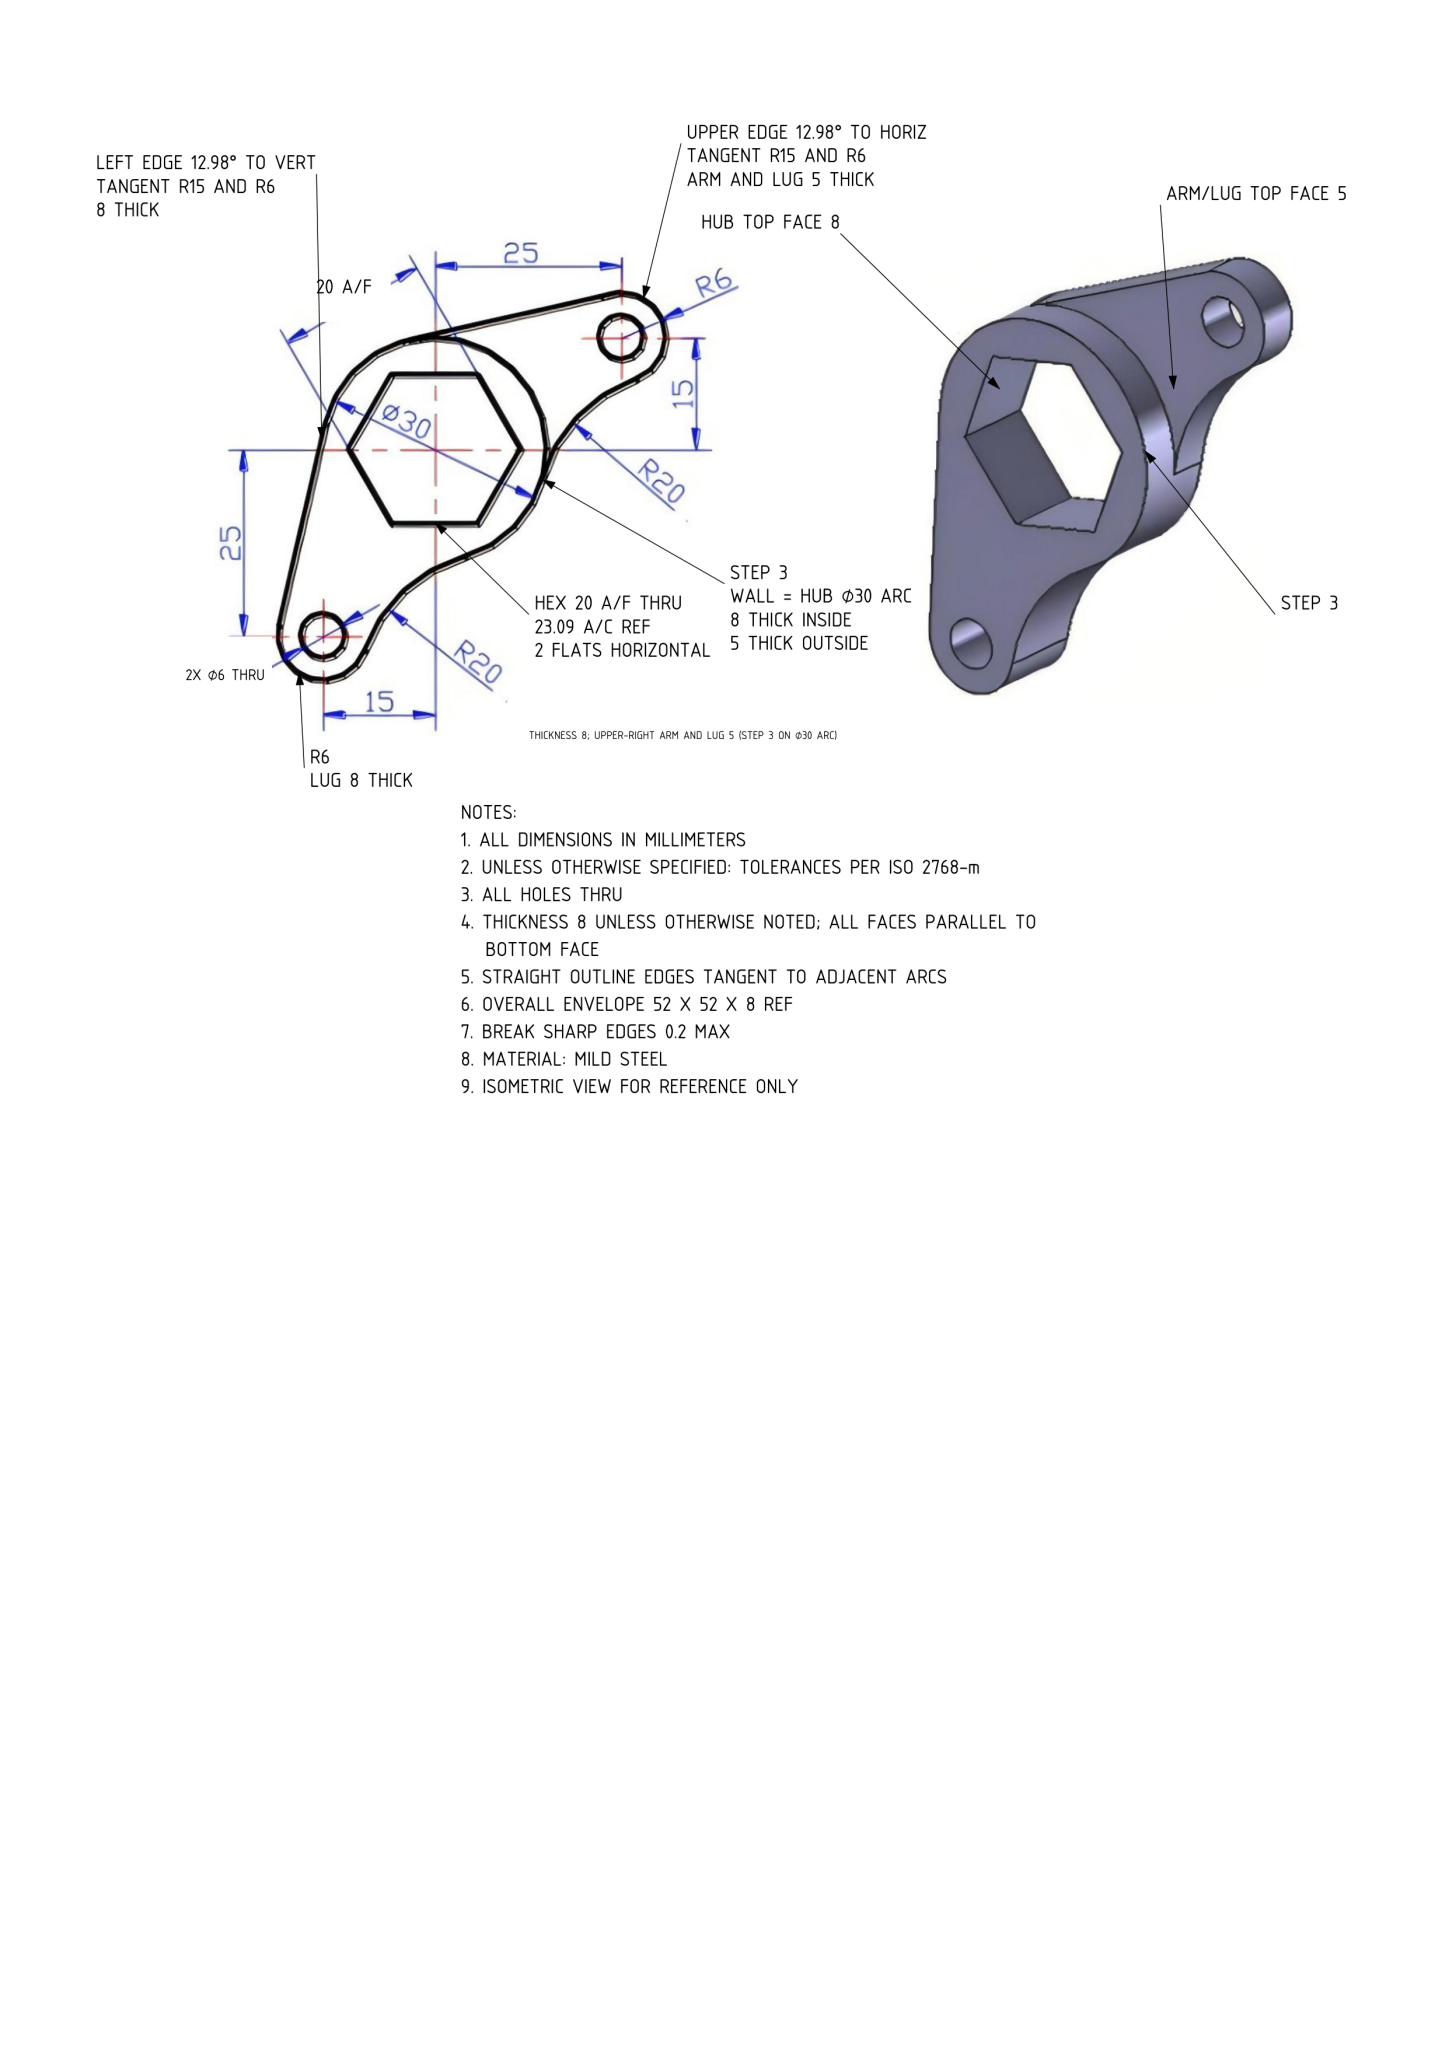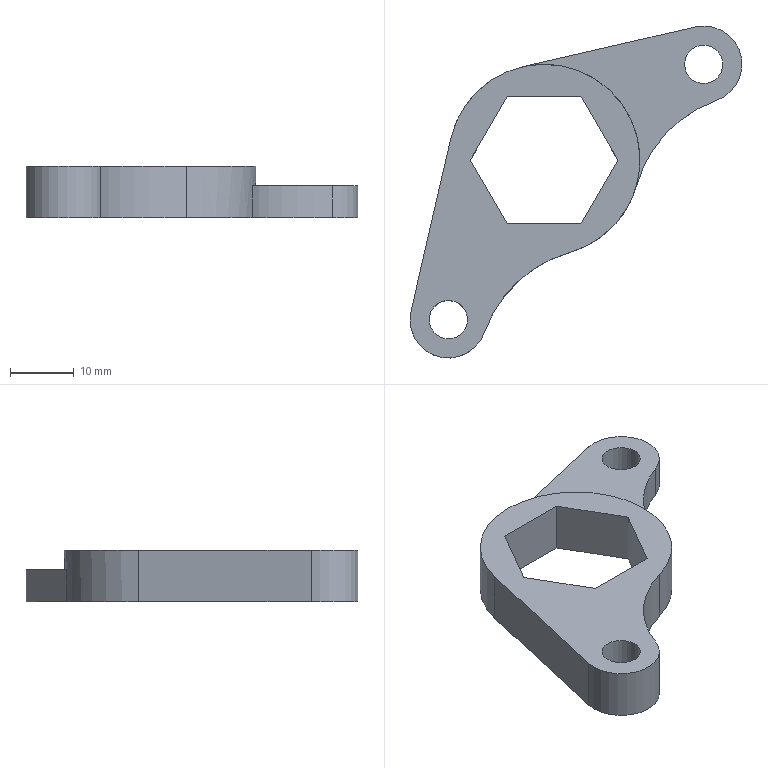Part | NX | mm | 1 solid | 18 faces | box 52 x 52 x 8 mm | volume 6324 mm3 | plane 11 | cylinder 7 | commonest cylinder face diameters 40 x2 12 x2 6 x2 30 x1
STEP:
#1=CARTESIAN_POINT('',(0.,0.,0.));
#2=DIRECTION('',(0.,0.,1.));
#3=DIRECTION('',(1.,0.,0.));
#4=AXIS2_PLACEMENT_3D('',#1,#2,#3);
#5=(LENGTH_UNIT()NAMED_UNIT(*)SI_UNIT(.MILLI.,.METRE.));
#6=UNCERTAINTY_MEASURE_WITH_UNIT(LENGTH_MEASURE(0.00002),#5,'','');
#7=(NAMED_UNIT(*)PLANE_ANGLE_UNIT()SI_UNIT($,.RADIAN.));
#8=PLANE_ANGLE_MEASURE_WITH_UNIT(PLANE_ANGLE_MEASURE(0.01745),#7);
#9=DIMENSIONAL_EXPONENTS(0.,0.,0.,0.,0.,0.,0.);
#10=(CONVERSION_BASED_UNIT('',#8)NAMED_UNIT(#9)PLANE_ANGLE_UNIT());
#11=(NAMED_UNIT(*)SI_UNIT($,.STERADIAN.)SOLID_ANGLE_UNIT());
#12=(GEOMETRIC_REPRESENTATION_CONTEXT(3)GLOBAL_UNCERTAINTY_ASSIGNED_CONTEXT((#6))GLOBAL_UNIT_ASSIGNED_CONTEXT((#5,#10,#11))REPRESENTATION_CONTEXT('',''));
#13=SHAPE_REPRESENTATION('',(#4),#12);
#14=CARTESIAN_POINT('',(-11.547,0.,0.));
#15=VERTEX_POINT('',#14);
#16=CARTESIAN_POINT('',(-5.774,-10.,0.));
#17=VERTEX_POINT('',#16);
#18=CARTESIAN_POINT('',(-11.547,0.,0.));
#19=DIRECTION('',(0.5,-0.866,0.));
#20=VECTOR('',#19,1.);
#21=LINE('',#18,#20);
#22=EDGE_CURVE('',#15,#17,#21,.T.);
#23=ORIENTED_EDGE('',*,*,#22,.F.);
#24=CARTESIAN_POINT('',(-11.547,0.,8.));
#25=VERTEX_POINT('',#24);
#26=CARTESIAN_POINT('',(-11.547,0.,8.));
#27=DIRECTION('',(0.,0.,-1.));
#28=VECTOR('',#27,1.);
#29=LINE('',#26,#28);
#30=EDGE_CURVE('',#25,#15,#29,.T.);
#31=ORIENTED_EDGE('',*,*,#30,.F.);
#32=CARTESIAN_POINT('',(-5.774,-10.,8.));
#33=VERTEX_POINT('',#32);
#34=CARTESIAN_POINT('',(-11.547,0.,8.));
#35=DIRECTION('',(0.5,-0.866,0.));
#36=VECTOR('',#35,1.);
#37=LINE('',#34,#36);
#38=EDGE_CURVE('',#25,#33,#37,.T.);
#39=ORIENTED_EDGE('',*,*,#38,.T.);
#40=CARTESIAN_POINT('',(-5.774,-10.,8.));
#41=DIRECTION('',(0.,0.,-1.));
#42=VECTOR('',#41,1.);
#43=LINE('',#40,#42);
#44=EDGE_CURVE('',#33,#17,#43,.T.);
#45=ORIENTED_EDGE('',*,*,#44,.T.);
#46=EDGE_LOOP('',(#23,#31,#39,#45));
#47=FACE_OUTER_BOUND('',#46,.T.);
#48=CARTESIAN_POINT('',(-11.547,0.,8.));
#49=DIRECTION('',(0.866,0.5,0.));
#50=DIRECTION('',(-0.5,0.866,0.));
#51=AXIS2_PLACEMENT_3D('',#48,#49,#50);
#52=PLANE('',#51);
#53=ADVANCED_FACE('',(#47),#52,.T.);
#54=CARTESIAN_POINT('',(5.774,-10.,0.));
#55=VERTEX_POINT('',#54);
#56=CARTESIAN_POINT('',(-5.774,-10.,0.));
#57=DIRECTION('',(1.,-0.,0.));
#58=VECTOR('',#57,1.);
#59=LINE('',#56,#58);
#60=EDGE_CURVE('',#17,#55,#59,.T.);
#61=ORIENTED_EDGE('',*,*,#60,.F.);
#62=ORIENTED_EDGE('',*,*,#44,.F.);
#63=CARTESIAN_POINT('',(5.774,-10.,8.));
#64=VERTEX_POINT('',#63);
#65=CARTESIAN_POINT('',(-5.774,-10.,8.));
#66=DIRECTION('',(1.,-0.,0.));
#67=VECTOR('',#66,1.);
#68=LINE('',#65,#67);
#69=EDGE_CURVE('',#33,#64,#68,.T.);
#70=ORIENTED_EDGE('',*,*,#69,.T.);
#71=CARTESIAN_POINT('',(5.774,-10.,8.));
#72=DIRECTION('',(0.,0.,-1.));
#73=VECTOR('',#72,1.);
#74=LINE('',#71,#73);
#75=EDGE_CURVE('',#64,#55,#74,.T.);
#76=ORIENTED_EDGE('',*,*,#75,.T.);
#77=EDGE_LOOP('',(#61,#62,#70,#76));
#78=FACE_OUTER_BOUND('',#77,.T.);
#79=CARTESIAN_POINT('',(-5.774,-10.,8.));
#80=DIRECTION('',(0.,1.,0.));
#81=DIRECTION('',(-1.,0.,0.));
#82=AXIS2_PLACEMENT_3D('',#79,#80,#81);
#83=PLANE('',#82);
#84=ADVANCED_FACE('',(#78),#83,.T.);
#85=CARTESIAN_POINT('',(11.547,-0.,0.));
#86=VERTEX_POINT('',#85);
#87=CARTESIAN_POINT('',(5.774,-10.,0.));
#88=DIRECTION('',(0.5,0.866,0.));
#89=VECTOR('',#88,1.);
#90=LINE('',#87,#89);
#91=EDGE_CURVE('',#55,#86,#90,.T.);
#92=ORIENTED_EDGE('',*,*,#91,.F.);
#93=ORIENTED_EDGE('',*,*,#75,.F.);
#94=CARTESIAN_POINT('',(11.547,-0.,8.));
#95=VERTEX_POINT('',#94);
#96=CARTESIAN_POINT('',(5.774,-10.,8.));
#97=DIRECTION('',(0.5,0.866,0.));
#98=VECTOR('',#97,1.);
#99=LINE('',#96,#98);
#100=EDGE_CURVE('',#64,#95,#99,.T.);
#101=ORIENTED_EDGE('',*,*,#100,.T.);
#102=CARTESIAN_POINT('',(11.547,-0.,8.));
#103=DIRECTION('',(0.,0.,-1.));
#104=VECTOR('',#103,1.);
#105=LINE('',#102,#104);
#106=EDGE_CURVE('',#95,#86,#105,.T.);
#107=ORIENTED_EDGE('',*,*,#106,.T.);
#108=EDGE_LOOP('',(#92,#93,#101,#107));
#109=FACE_OUTER_BOUND('',#108,.T.);
#110=CARTESIAN_POINT('',(5.774,-10.,8.));
#111=DIRECTION('',(-0.866,0.5,0.));
#112=DIRECTION('',(-0.5,-0.866,0.));
#113=AXIS2_PLACEMENT_3D('',#110,#111,#112);
#114=PLANE('',#113);
#115=ADVANCED_FACE('',(#109),#114,.T.);
#116=CARTESIAN_POINT('',(5.774,10.,0.));
#117=VERTEX_POINT('',#116);
#118=CARTESIAN_POINT('',(11.547,-0.,0.));
#119=DIRECTION('',(-0.5,0.866,0.));
#120=VECTOR('',#119,1.);
#121=LINE('',#118,#120);
#122=EDGE_CURVE('',#86,#117,#121,.T.);
#123=ORIENTED_EDGE('',*,*,#122,.F.);
#124=ORIENTED_EDGE('',*,*,#106,.F.);
#125=CARTESIAN_POINT('',(5.774,10.,8.));
#126=VERTEX_POINT('',#125);
#127=CARTESIAN_POINT('',(11.547,-0.,8.));
#128=DIRECTION('',(-0.5,0.866,0.));
#129=VECTOR('',#128,1.);
#130=LINE('',#127,#129);
#131=EDGE_CURVE('',#95,#126,#130,.T.);
#132=ORIENTED_EDGE('',*,*,#131,.T.);
#133=CARTESIAN_POINT('',(5.774,10.,8.));
#134=DIRECTION('',(0.,0.,-1.));
#135=VECTOR('',#134,1.);
#136=LINE('',#133,#135);
#137=EDGE_CURVE('',#126,#117,#136,.T.);
#138=ORIENTED_EDGE('',*,*,#137,.T.);
#139=EDGE_LOOP('',(#123,#124,#132,#138));
#140=FACE_OUTER_BOUND('',#139,.T.);
#141=CARTESIAN_POINT('',(11.547,-0.,8.));
#142=DIRECTION('',(-0.866,-0.5,0.));
#143=DIRECTION('',(0.5,-0.866,0.));
#144=AXIS2_PLACEMENT_3D('',#141,#142,#143);
#145=PLANE('',#144);
#146=ADVANCED_FACE('',(#140),#145,.T.);
#147=CARTESIAN_POINT('',(-5.774,10.,0.));
#148=VERTEX_POINT('',#147);
#149=CARTESIAN_POINT('',(5.774,10.,0.));
#150=DIRECTION('',(-1.,0.,0.));
#151=VECTOR('',#150,1.);
#152=LINE('',#149,#151);
#153=EDGE_CURVE('',#117,#148,#152,.T.);
#154=ORIENTED_EDGE('',*,*,#153,.F.);
#155=ORIENTED_EDGE('',*,*,#137,.F.);
#156=CARTESIAN_POINT('',(-5.774,10.,8.));
#157=VERTEX_POINT('',#156);
#158=CARTESIAN_POINT('',(5.774,10.,8.));
#159=DIRECTION('',(-1.,0.,0.));
#160=VECTOR('',#159,1.);
#161=LINE('',#158,#160);
#162=EDGE_CURVE('',#126,#157,#161,.T.);
#163=ORIENTED_EDGE('',*,*,#162,.T.);
#164=CARTESIAN_POINT('',(-5.774,10.,8.));
#165=DIRECTION('',(0.,0.,-1.));
#166=VECTOR('',#165,1.);
#167=LINE('',#164,#166);
#168=EDGE_CURVE('',#157,#148,#167,.T.);
#169=ORIENTED_EDGE('',*,*,#168,.T.);
#170=EDGE_LOOP('',(#154,#155,#163,#169));
#171=FACE_OUTER_BOUND('',#170,.T.);
#172=CARTESIAN_POINT('',(5.774,10.,8.));
#173=DIRECTION('',(-0.,-1.,0.));
#174=DIRECTION('',(1.,-0.,0.));
#175=AXIS2_PLACEMENT_3D('',#172,#173,#174);
#176=PLANE('',#175);
#177=ADVANCED_FACE('',(#171),#176,.T.);
#178=CARTESIAN_POINT('',(4.074,-14.436,0.));
#179=VERTEX_POINT('',#178);
#180=CARTESIAN_POINT('',(-9.345,-27.004,0.));
#181=VERTEX_POINT('',#180);
#182=CARTESIAN_POINT('',(9.507,-33.684,0.));
#183=DIRECTION('',(0.,0.,1.));
#184=DIRECTION('',(1.,0.,0.));
#185=AXIS2_PLACEMENT_3D('',#182,#183,#184);
#186=CIRCLE('',#185,20.);
#187=EDGE_CURVE('',#179,#181,#186,.T.);
#188=ORIENTED_EDGE('',*,*,#187,.F.);
#189=CARTESIAN_POINT('',(4.074,-14.436,8.));
#190=VERTEX_POINT('',#189);
#191=CARTESIAN_POINT('',(4.074,-14.436,8.));
#192=DIRECTION('',(0.,0.,-1.));
#193=VECTOR('',#192,1.);
#194=LINE('',#191,#193);
#195=EDGE_CURVE('',#190,#179,#194,.T.);
#196=ORIENTED_EDGE('',*,*,#195,.F.);
#197=CARTESIAN_POINT('',(-9.345,-27.004,8.));
#198=VERTEX_POINT('',#197);
#199=CARTESIAN_POINT('',(9.507,-33.684,8.));
#200=DIRECTION('',(0.,0.,1.));
#201=DIRECTION('',(1.,0.,0.));
#202=AXIS2_PLACEMENT_3D('',#199,#200,#201);
#203=CIRCLE('',#202,20.);
#204=EDGE_CURVE('',#190,#198,#203,.T.);
#205=ORIENTED_EDGE('',*,*,#204,.T.);
#206=CARTESIAN_POINT('',(-9.345,-27.004,8.));
#207=DIRECTION('',(0.,0.,-1.));
#208=VECTOR('',#207,1.);
#209=LINE('',#206,#208);
#210=EDGE_CURVE('',#198,#181,#209,.T.);
#211=ORIENTED_EDGE('',*,*,#210,.T.);
#212=EDGE_LOOP('',(#188,#196,#205,#211));
#213=FACE_OUTER_BOUND('',#212,.T.);
#214=CARTESIAN_POINT('',(9.507,-33.684,8.));
#215=DIRECTION('',(0.,0.,-1.));
#216=DIRECTION('',(-1.,0.,0.));
#217=AXIS2_PLACEMENT_3D('',#214,#215,#216);
#218=CYLINDRICAL_SURFACE('',#217,20.);
#219=ADVANCED_FACE('',(#213),#218,.F.);
#220=CARTESIAN_POINT('',(-20.847,-23.652,0.));
#221=VERTEX_POINT('',#220);
#222=CARTESIAN_POINT('',(-15.,-25.,0.));
#223=DIRECTION('',(0.,0.,-1.));
#224=DIRECTION('',(1.,0.,0.));
#225=AXIS2_PLACEMENT_3D('',#222,#223,#224);
#226=CIRCLE('',#225,6.);
#227=EDGE_CURVE('',#181,#221,#226,.T.);
#228=ORIENTED_EDGE('',*,*,#227,.F.);
#229=ORIENTED_EDGE('',*,*,#210,.F.);
#230=CARTESIAN_POINT('',(-20.847,-23.652,8.));
#231=VERTEX_POINT('',#230);
#232=CARTESIAN_POINT('',(-15.,-25.,8.));
#233=DIRECTION('',(0.,0.,-1.));
#234=DIRECTION('',(1.,0.,0.));
#235=AXIS2_PLACEMENT_3D('',#232,#233,#234);
#236=CIRCLE('',#235,6.);
#237=EDGE_CURVE('',#198,#231,#236,.T.);
#238=ORIENTED_EDGE('',*,*,#237,.T.);
#239=CARTESIAN_POINT('',(-20.847,-23.652,8.));
#240=DIRECTION('',(0.,0.,-1.));
#241=VECTOR('',#240,1.);
#242=LINE('',#239,#241);
#243=EDGE_CURVE('',#231,#221,#242,.T.);
#244=ORIENTED_EDGE('',*,*,#243,.T.);
#245=EDGE_LOOP('',(#228,#229,#238,#244));
#246=FACE_OUTER_BOUND('',#245,.T.);
#247=CARTESIAN_POINT('',(-15.,-25.,8.));
#248=DIRECTION('',(0.,0.,-1.));
#249=DIRECTION('',(-1.,0.,0.));
#250=AXIS2_PLACEMENT_3D('',#247,#248,#249);
#251=CYLINDRICAL_SURFACE('',#250,6.);
#252=ADVANCED_FACE('',(#246),#251,.T.);
#253=CARTESIAN_POINT('',(-14.617,3.37,0.));
#254=VERTEX_POINT('',#253);
#255=CARTESIAN_POINT('',(-20.847,-23.652,0.));
#256=DIRECTION('',(0.2247,0.9744,0.));
#257=VECTOR('',#256,1.);
#258=LINE('',#255,#257);
#259=EDGE_CURVE('',#221,#254,#258,.T.);
#260=ORIENTED_EDGE('',*,*,#259,.F.);
#261=ORIENTED_EDGE('',*,*,#243,.F.);
#262=CARTESIAN_POINT('',(-14.617,3.37,8.));
#263=VERTEX_POINT('',#262);
#264=CARTESIAN_POINT('',(-20.847,-23.652,8.));
#265=DIRECTION('',(0.2247,0.9744,0.));
#266=VECTOR('',#265,1.);
#267=LINE('',#264,#266);
#268=EDGE_CURVE('',#231,#263,#267,.T.);
#269=ORIENTED_EDGE('',*,*,#268,.T.);
#270=CARTESIAN_POINT('',(-14.617,3.37,8.));
#271=DIRECTION('',(0.,0.,-1.));
#272=VECTOR('',#271,1.);
#273=LINE('',#270,#272);
#274=EDGE_CURVE('',#263,#254,#273,.T.);
#275=ORIENTED_EDGE('',*,*,#274,.T.);
#276=EDGE_LOOP('',(#260,#261,#269,#275));
#277=FACE_OUTER_BOUND('',#276,.T.);
#278=CARTESIAN_POINT('',(-20.847,-23.652,8.));
#279=DIRECTION('',(-0.9744,0.2247,0.));
#280=DIRECTION('',(-0.2247,-0.9744,0.));
#281=AXIS2_PLACEMENT_3D('',#278,#279,#280);
#282=PLANE('',#281);
#283=ADVANCED_FACE('',(#277),#282,.T.);
#284=CARTESIAN_POINT('',(-5.774,10.,0.));
#285=DIRECTION('',(-0.5,-0.866,0.));
#286=VECTOR('',#285,1.);
#287=LINE('',#284,#286);
#288=EDGE_CURVE('',#148,#15,#287,.T.);
#289=ORIENTED_EDGE('',*,*,#288,.F.);
#290=ORIENTED_EDGE('',*,*,#168,.F.);
#291=CARTESIAN_POINT('',(-5.774,10.,8.));
#292=DIRECTION('',(-0.5,-0.866,0.));
#293=VECTOR('',#292,1.);
#294=LINE('',#291,#293);
#295=EDGE_CURVE('',#157,#25,#294,.T.);
#296=ORIENTED_EDGE('',*,*,#295,.T.);
#297=ORIENTED_EDGE('',*,*,#30,.T.);
#298=EDGE_LOOP('',(#289,#290,#296,#297));
#299=FACE_OUTER_BOUND('',#298,.T.);
#300=CARTESIAN_POINT('',(-5.774,10.,8.));
#301=DIRECTION('',(0.866,-0.5,0.));
#302=DIRECTION('',(0.5,0.866,0.));
#303=AXIS2_PLACEMENT_3D('',#300,#301,#302);
#304=PLANE('',#303);
#305=ADVANCED_FACE('',(#299),#304,.T.);
#306=CARTESIAN_POINT('',(14.436,-4.074,5.));
#307=VERTEX_POINT('',#306);
#308=CARTESIAN_POINT('',(14.436,-4.074,0.));
#309=VERTEX_POINT('',#308);
#310=CARTESIAN_POINT('',(14.436,-4.074,5.));
#311=DIRECTION('',(0.,0.,-1.));
#312=VECTOR('',#311,1.);
#313=LINE('',#310,#312);
#314=EDGE_CURVE('',#307,#309,#313,.T.);
#315=ORIENTED_EDGE('',*,*,#314,.F.);
#316=CARTESIAN_POINT('',(-3.37,14.617,5.));
#317=VERTEX_POINT('',#316);
#318=CARTESIAN_POINT('',(0.,0.,5.));
#319=DIRECTION('',(0.,0.,-1.));
#320=DIRECTION('',(1.,0.,0.));
#321=AXIS2_PLACEMENT_3D('',#318,#319,#320);
#322=CIRCLE('',#321,15.);
#323=EDGE_CURVE('',#317,#307,#322,.T.);
#324=ORIENTED_EDGE('',*,*,#323,.F.);
#325=CARTESIAN_POINT('',(-3.37,14.617,0.));
#326=VERTEX_POINT('',#325);
#327=CARTESIAN_POINT('',(-3.37,14.617,5.));
#328=DIRECTION('',(0.,0.,-1.));
#329=VECTOR('',#328,1.);
#330=LINE('',#327,#329);
#331=EDGE_CURVE('',#317,#326,#330,.T.);
#332=ORIENTED_EDGE('',*,*,#331,.T.);
#333=CARTESIAN_POINT('',(0.,0.,0.));
#334=DIRECTION('',(0.,0.,-1.));
#335=DIRECTION('',(1.,0.,0.));
#336=AXIS2_PLACEMENT_3D('',#333,#334,#335);
#337=CIRCLE('',#336,15.);
#338=EDGE_CURVE('',#254,#326,#337,.T.);
#339=ORIENTED_EDGE('',*,*,#338,.F.);
#340=ORIENTED_EDGE('',*,*,#274,.F.);
#341=CARTESIAN_POINT('',(0.,0.,8.));
#342=DIRECTION('',(0.,0.,-1.));
#343=DIRECTION('',(1.,0.,0.));
#344=AXIS2_PLACEMENT_3D('',#341,#342,#343);
#345=CIRCLE('',#344,15.);
#346=EDGE_CURVE('',#263,#190,#345,.T.);
#347=ORIENTED_EDGE('',*,*,#346,.T.);
#348=ORIENTED_EDGE('',*,*,#195,.T.);
#349=CARTESIAN_POINT('',(0.,0.,0.));
#350=DIRECTION('',(0.,0.,-1.));
#351=DIRECTION('',(1.,0.,0.));
#352=AXIS2_PLACEMENT_3D('',#349,#350,#351);
#353=CIRCLE('',#352,15.);
#354=EDGE_CURVE('',#309,#179,#353,.T.);
#355=ORIENTED_EDGE('',*,*,#354,.F.);
#356=EDGE_LOOP('',(#315,#324,#332,#339,#340,#347,#348,#355));
#357=FACE_OUTER_BOUND('',#356,.T.);
#358=CARTESIAN_POINT('',(0.,0.,8.));
#359=DIRECTION('',(0.,0.,-1.));
#360=DIRECTION('',(-1.,0.,0.));
#361=AXIS2_PLACEMENT_3D('',#358,#359,#360);
#362=CYLINDRICAL_SURFACE('',#361,15.);
#363=ADVANCED_FACE('',(#357),#362,.T.);
#364=CARTESIAN_POINT('',(-12.,-25.,8.));
#365=VERTEX_POINT('',#364);
#366=CARTESIAN_POINT('',(-15.,-25.,8.));
#367=DIRECTION('',(0.,0.,1.));
#368=DIRECTION('',(1.,0.,0.));
#369=AXIS2_PLACEMENT_3D('',#366,#367,#368);
#370=CIRCLE('',#369,3.);
#371=EDGE_CURVE('',#365,#365,#370,.T.);
#372=ORIENTED_EDGE('',*,*,#371,.T.);
#373=EDGE_LOOP('',(#372));
#374=FACE_BOUND('',#373,.T.);
#375=CARTESIAN_POINT('',(-12.,-25.,0.));
#376=VERTEX_POINT('',#375);
#377=CARTESIAN_POINT('',(-15.,-25.,0.));
#378=DIRECTION('',(0.,0.,1.));
#379=DIRECTION('',(1.,0.,0.));
#380=AXIS2_PLACEMENT_3D('',#377,#378,#379);
#381=CIRCLE('',#380,3.);
#382=EDGE_CURVE('',#376,#376,#381,.T.);
#383=ORIENTED_EDGE('',*,*,#382,.F.);
#384=EDGE_LOOP('',(#383));
#385=FACE_BOUND('',#384,.T.);
#386=CARTESIAN_POINT('',(-15.,-25.,8.));
#387=DIRECTION('',(0.,0.,-1.));
#388=DIRECTION('',(-1.,0.,0.));
#389=AXIS2_PLACEMENT_3D('',#386,#387,#388);
#390=CYLINDRICAL_SURFACE('',#389,3.);
#391=ADVANCED_FACE('',(#374,#385),#390,.F.);
#392=ORIENTED_EDGE('',*,*,#204,.F.);
#393=ORIENTED_EDGE('',*,*,#346,.F.);
#394=ORIENTED_EDGE('',*,*,#268,.F.);
#395=ORIENTED_EDGE('',*,*,#237,.F.);
#396=EDGE_LOOP('',(#392,#393,#394,#395));
#397=FACE_BOUND('',#396,.T.);
#398=ORIENTED_EDGE('',*,*,#38,.F.);
#399=ORIENTED_EDGE('',*,*,#295,.F.);
#400=ORIENTED_EDGE('',*,*,#162,.F.);
#401=ORIENTED_EDGE('',*,*,#131,.F.);
#402=ORIENTED_EDGE('',*,*,#100,.F.);
#403=ORIENTED_EDGE('',*,*,#69,.F.);
#404=EDGE_LOOP('',(#398,#399,#400,#401,#402,#403));
#405=FACE_BOUND('',#404,.T.);
#406=ORIENTED_EDGE('',*,*,#371,.F.);
#407=EDGE_LOOP('',(#406));
#408=FACE_BOUND('',#407,.T.);
#409=CARTESIAN_POINT('',(9.507,-33.684,8.));
#410=DIRECTION('',(0.,0.,1.));
#411=DIRECTION('',(1.,0.,0.));
#412=AXIS2_PLACEMENT_3D('',#409,#410,#411);
#413=PLANE('',#412);
#414=ADVANCED_FACE('',(#397,#405,#408),#413,.T.);
#415=ORIENTED_EDGE('',*,*,#187,.T.);
#416=ORIENTED_EDGE('',*,*,#227,.T.);
#417=ORIENTED_EDGE('',*,*,#259,.T.);
#418=ORIENTED_EDGE('',*,*,#338,.T.);
#419=CARTESIAN_POINT('',(23.652,20.847,0.));
#420=VERTEX_POINT('',#419);
#421=CARTESIAN_POINT('',(23.652,20.847,0.));
#422=DIRECTION('',(-0.9744,-0.2247,0.));
#423=VECTOR('',#422,1.);
#424=LINE('',#421,#423);
#425=EDGE_CURVE('',#420,#326,#424,.T.);
#426=ORIENTED_EDGE('',*,*,#425,.F.);
#427=CARTESIAN_POINT('',(27.004,9.345,0.));
#428=VERTEX_POINT('',#427);
#429=CARTESIAN_POINT('',(25.,15.,0.));
#430=DIRECTION('',(0.,0.,1.));
#431=DIRECTION('',(1.,0.,0.));
#432=AXIS2_PLACEMENT_3D('',#429,#430,#431);
#433=CIRCLE('',#432,6.);
#434=EDGE_CURVE('',#428,#420,#433,.T.);
#435=ORIENTED_EDGE('',*,*,#434,.F.);
#436=CARTESIAN_POINT('',(33.684,-9.507,0.));
#437=DIRECTION('',(0.,0.,-1.));
#438=DIRECTION('',(1.,0.,0.));
#439=AXIS2_PLACEMENT_3D('',#436,#437,#438);
#440=CIRCLE('',#439,20.);
#441=EDGE_CURVE('',#309,#428,#440,.T.);
#442=ORIENTED_EDGE('',*,*,#441,.F.);
#443=ORIENTED_EDGE('',*,*,#354,.T.);
#444=EDGE_LOOP('',(#415,#416,#417,#418,#426,#435,#442,#443));
#445=FACE_BOUND('',#444,.T.);
#446=ORIENTED_EDGE('',*,*,#22,.T.);
#447=ORIENTED_EDGE('',*,*,#60,.T.);
#448=ORIENTED_EDGE('',*,*,#91,.T.);
#449=ORIENTED_EDGE('',*,*,#122,.T.);
#450=ORIENTED_EDGE('',*,*,#153,.T.);
#451=ORIENTED_EDGE('',*,*,#288,.T.);
#452=EDGE_LOOP('',(#446,#447,#448,#449,#450,#451));
#453=FACE_BOUND('',#452,.T.);
#454=ORIENTED_EDGE('',*,*,#382,.T.);
#455=EDGE_LOOP('',(#454));
#456=FACE_BOUND('',#455,.T.);
#457=CARTESIAN_POINT('',(28.,15.,0.));
#458=VERTEX_POINT('',#457);
#459=CARTESIAN_POINT('',(25.,15.,0.));
#460=DIRECTION('',(0.,0.,1.));
#461=DIRECTION('',(1.,0.,0.));
#462=AXIS2_PLACEMENT_3D('',#459,#460,#461);
#463=CIRCLE('',#462,3.);
#464=EDGE_CURVE('',#458,#458,#463,.T.);
#465=ORIENTED_EDGE('',*,*,#464,.T.);
#466=EDGE_LOOP('',(#465));
#467=FACE_BOUND('',#466,.T.);
#468=CARTESIAN_POINT('',(9.507,-33.684,0.));
#469=DIRECTION('',(0.,0.,1.));
#470=DIRECTION('',(1.,0.,0.));
#471=AXIS2_PLACEMENT_3D('',#468,#469,#470);
#472=PLANE('',#471);
#473=ADVANCED_FACE('',(#445,#453,#456,#467),#472,.F.);
#474=ORIENTED_EDGE('',*,*,#441,.T.);
#475=CARTESIAN_POINT('',(27.004,9.345,5.));
#476=VERTEX_POINT('',#475);
#477=CARTESIAN_POINT('',(27.004,9.345,5.));
#478=DIRECTION('',(0.,0.,-1.));
#479=VECTOR('',#478,1.);
#480=LINE('',#477,#479);
#481=EDGE_CURVE('',#476,#428,#480,.T.);
#482=ORIENTED_EDGE('',*,*,#481,.F.);
#483=CARTESIAN_POINT('',(33.684,-9.507,5.));
#484=DIRECTION('',(0.,0.,-1.));
#485=DIRECTION('',(1.,0.,0.));
#486=AXIS2_PLACEMENT_3D('',#483,#484,#485);
#487=CIRCLE('',#486,20.);
#488=EDGE_CURVE('',#307,#476,#487,.T.);
#489=ORIENTED_EDGE('',*,*,#488,.F.);
#490=ORIENTED_EDGE('',*,*,#314,.T.);
#491=EDGE_LOOP('',(#474,#482,#489,#490));
#492=FACE_OUTER_BOUND('',#491,.T.);
#493=CARTESIAN_POINT('',(33.684,-9.507,5.));
#494=DIRECTION('',(0.,0.,-1.));
#495=DIRECTION('',(-1.,0.,0.));
#496=AXIS2_PLACEMENT_3D('',#493,#494,#495);
#497=CYLINDRICAL_SURFACE('',#496,20.);
#498=ADVANCED_FACE('',(#492),#497,.F.);
#499=ORIENTED_EDGE('',*,*,#434,.T.);
#500=CARTESIAN_POINT('',(23.652,20.847,5.));
#501=VERTEX_POINT('',#500);
#502=CARTESIAN_POINT('',(23.652,20.847,5.));
#503=DIRECTION('',(0.,0.,-1.));
#504=VECTOR('',#503,1.);
#505=LINE('',#502,#504);
#506=EDGE_CURVE('',#501,#420,#505,.T.);
#507=ORIENTED_EDGE('',*,*,#506,.F.);
#508=CARTESIAN_POINT('',(25.,15.,5.));
#509=DIRECTION('',(0.,0.,1.));
#510=DIRECTION('',(1.,0.,0.));
#511=AXIS2_PLACEMENT_3D('',#508,#509,#510);
#512=CIRCLE('',#511,6.);
#513=EDGE_CURVE('',#476,#501,#512,.T.);
#514=ORIENTED_EDGE('',*,*,#513,.F.);
#515=ORIENTED_EDGE('',*,*,#481,.T.);
#516=EDGE_LOOP('',(#499,#507,#514,#515));
#517=FACE_OUTER_BOUND('',#516,.T.);
#518=CARTESIAN_POINT('',(25.,15.,5.));
#519=DIRECTION('',(0.,0.,-1.));
#520=DIRECTION('',(-1.,0.,0.));
#521=AXIS2_PLACEMENT_3D('',#518,#519,#520);
#522=CYLINDRICAL_SURFACE('',#521,6.);
#523=ADVANCED_FACE('',(#517),#522,.T.);
#524=ORIENTED_EDGE('',*,*,#425,.T.);
#525=ORIENTED_EDGE('',*,*,#331,.F.);
#526=CARTESIAN_POINT('',(23.652,20.847,5.));
#527=DIRECTION('',(-0.9744,-0.2247,0.));
#528=VECTOR('',#527,1.);
#529=LINE('',#526,#528);
#530=EDGE_CURVE('',#501,#317,#529,.T.);
#531=ORIENTED_EDGE('',*,*,#530,.F.);
#532=ORIENTED_EDGE('',*,*,#506,.T.);
#533=EDGE_LOOP('',(#524,#525,#531,#532));
#534=FACE_OUTER_BOUND('',#533,.T.);
#535=CARTESIAN_POINT('',(23.652,20.847,5.));
#536=DIRECTION('',(0.2247,-0.9744,0.));
#537=DIRECTION('',(0.9744,0.2247,0.));
#538=AXIS2_PLACEMENT_3D('',#535,#536,#537);
#539=PLANE('',#538);
#540=ADVANCED_FACE('',(#534),#539,.F.);
#541=CARTESIAN_POINT('',(28.,15.,5.));
#542=VERTEX_POINT('',#541);
#543=CARTESIAN_POINT('',(25.,15.,5.));
#544=DIRECTION('',(0.,0.,1.));
#545=DIRECTION('',(1.,0.,0.));
#546=AXIS2_PLACEMENT_3D('',#543,#544,#545);
#547=CIRCLE('',#546,3.);
#548=EDGE_CURVE('',#542,#542,#547,.T.);
#549=ORIENTED_EDGE('',*,*,#548,.T.);
#550=EDGE_LOOP('',(#549));
#551=FACE_BOUND('',#550,.T.);
#552=ORIENTED_EDGE('',*,*,#464,.F.);
#553=EDGE_LOOP('',(#552));
#554=FACE_BOUND('',#553,.T.);
#555=CARTESIAN_POINT('',(25.,15.,5.));
#556=DIRECTION('',(0.,0.,-1.));
#557=DIRECTION('',(-1.,0.,0.));
#558=AXIS2_PLACEMENT_3D('',#555,#556,#557);
#559=CYLINDRICAL_SURFACE('',#558,3.);
#560=ADVANCED_FACE('',(#551,#554),#559,.F.);
#561=ORIENTED_EDGE('',*,*,#488,.T.);
#562=ORIENTED_EDGE('',*,*,#513,.T.);
#563=ORIENTED_EDGE('',*,*,#530,.T.);
#564=ORIENTED_EDGE('',*,*,#323,.T.);
#565=EDGE_LOOP('',(#561,#562,#563,#564));
#566=FACE_BOUND('',#565,.T.);
#567=ORIENTED_EDGE('',*,*,#548,.F.);
#568=EDGE_LOOP('',(#567));
#569=FACE_BOUND('',#568,.T.);
#570=CARTESIAN_POINT('',(33.684,-9.507,5.));
#571=DIRECTION('',(0.,0.,-1.));
#572=DIRECTION('',(-1.,0.,0.));
#573=AXIS2_PLACEMENT_3D('',#570,#571,#572);
#574=PLANE('',#573);
#575=ADVANCED_FACE('',(#566,#569),#574,.F.);
#576=CLOSED_SHELL('',(#53,#84,#115,#146,#177,#219,#252,#283,#305,#363,#391,#414,#473,#498,#523,#540,#560,#575));
#577=MANIFOLD_SOLID_BREP('',#576);
#578=ADVANCED_BREP_SHAPE_REPRESENTATION('',(#577),#12);
#579=SHAPE_REPRESENTATION_RELATIONSHIP('','',#13,#578);
#580=PRESENTATION_LAYER_ASSIGNMENT('','',(#577));
#581=COLOUR_RGB('',0.6784,0.6588,0.8314);
#582=FILL_AREA_STYLE_COLOUR('',#581);
#583=FILL_AREA_STYLE('',(#582));
#584=SURFACE_STYLE_FILL_AREA(#583);
#585=SURFACE_SIDE_STYLE('',(#584));
#586=SURFACE_STYLE_USAGE(.BOTH.,#585);
#587=PRESENTATION_STYLE_ASSIGNMENT((#586));
#588=STYLED_ITEM('',(#587),#577);
#589=MECHANICAL_DESIGN_GEOMETRIC_PRESENTATION_REPRESENTATION('',(#588),#12);